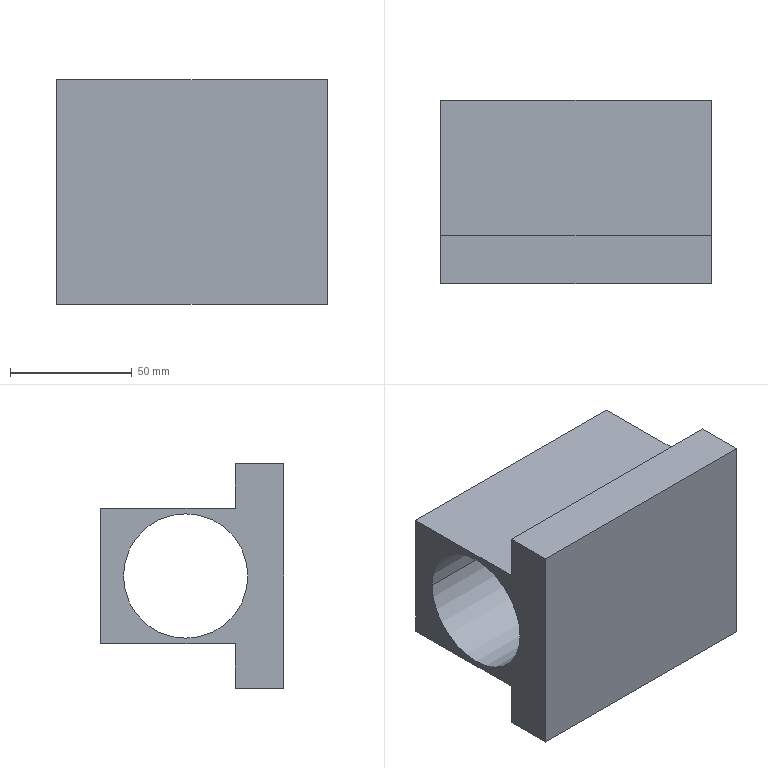Component | SolidWorks | ConnectingSeat-1 | 1 solid | 30 faces | box 111 x 75.24 x 92.14 mm | volume 314460 mm3 | plane 16 | cylinder 14 | commonest cylinder face diameters 8 x8 5.551 x4 51.14 x2
build123d program:
from build123d import *

# Parameters (mm, degrees)
BOSS_EXTRUDE1_DEPTH = 111
SKETCH4_R           = 18.564
CUT_EXTRUDE1_DEPTH  = 111
SKETCH5_W           = 55.24
SKETCH5_H           = 35.775
CUT_EXTRUDE2_DEPTH  = 171
SKETCH6_R           = 25.57
CUT_EXTRUDE3_DEPTH  = 115
SKETCH7_R           = 25.57
BOSS_EXTRUDE2_DEPTH = 111
SKETCH9_R           = 4
CUT_EXTRUDE4_DEPTH  = 13.5
SKETCH10_R          = 2.776
CUT_EXTRUDE5_DEPTH  = 13.5


with BuildPart() as part:
    # Sketch3 → Boss-Extrude1 (new body)
    with BuildSketch(Plane.ZY.offset(277)):
        Polygon((-20, -46.072), (-20, 46.072), (-0.1784, 46.072), (-0.1784, 27.887), (55.24, 27.887), (55.24, -27.887), (-0.1784, -27.887), (-0.1784, -46.072), align=None)
    extrude(amount=-BOSS_EXTRUDE1_DEPTH)

    # Sketch4 → Cut-Extrude1 (cut)
    with BuildSketch(Plane.ZY.offset(277)):
        with Locations((20.219, 0)):
            Circle(SKETCH4_R)
    extrude(amount=-CUT_EXTRUDE1_DEPTH, mode=Mode.SUBTRACT)

    # Sketch5 → Cut-Extrude2 (cut)
    with BuildSketch(Plane(origin=(-166, 0, 0), x_dir=(0, 0, -1), z_dir=(1, 0, 0))):
        with Locations((-17.62, 0)):
            Rectangle(SKETCH5_W, SKETCH5_H)
    extrude(amount=-CUT_EXTRUDE2_DEPTH, mode=Mode.SUBTRACT)

    # Sketch6 → Cut-Extrude3 (cut)
    with BuildSketch(Plane(origin=(-166, 0, 0), x_dir=(0, 0, -1), z_dir=(1, 0, 0))):
        with Locations((-20.219, 0)):
            Circle(SKETCH6_R)
    extrude(amount=-CUT_EXTRUDE3_DEPTH, mode=Mode.SUBTRACT)

    # Sketch7 → Boss-Extrude2 (add)
    with BuildSketch(Plane(origin=(-166, 0, 0), x_dir=(0, 0, -1), z_dir=(1, 0, 0))):
        Polygon((-55.24, 27.887), (-55.24, -27.887), (0.1784, -27.887), (0.1784, -46.072), (20, -46.072), (20, 46.072), (0.1784, 46.072), (0.1784, 27.887), align=None)
        with Locations((-20.219, 0)):
            Circle(SKETCH7_R, mode=Mode.SUBTRACT)
    extrude(amount=-BOSS_EXTRUDE2_DEPTH)

    # Sketch9 → Cut-Extrude4 (cut)
    with BuildSketch(Plane.XY.offset(-0.1784)):
        with Locations((-256.037, 36.566)):
            Circle(SKETCH9_R)
        with Locations((-186.382, 36.566)):
            Circle(SKETCH9_R)
        with Locations(Location((-186.382, -36.566, 0), (0, 0, 180))):
            Circle(SKETCH9_R)
        with Locations(Location((-256.037, -36.566, 0), (0, 0, 180))):
            Circle(SKETCH9_R)
    extrude(amount=-CUT_EXTRUDE4_DEPTH, mode=Mode.SUBTRACT)

    # Sketch10 → Cut-Extrude5 (cut)
    with BuildSketch(Plane.XY.offset(-0.1784)):
        with Locations((-221.326, 36.732)):
            Circle(SKETCH10_R)
        with Locations(Location((-221.326, -36.732, 0), (0, 0, 180))):
            Circle(SKETCH10_R)
    extrude(amount=-CUT_EXTRUDE5_DEPTH, mode=Mode.SUBTRACT)


solid = part.part

# Placed as in the assembly
solid = solid.moved(Location((0, 40, 0), (-90, 0, 0)))
STEP:
#1=CARTESIAN_POINT('',(-8.823,1.036,1.446));
#2=VERTEX_POINT('',#1);
#3=CARTESIAN_POINT('',(-8.604,1.036,1.446));
#4=VERTEX_POINT('',#3);
#5=CARTESIAN_POINT('',(-8.714,1.036,1.446));
#6=DIRECTION('',(0.,1.,0.));
#7=DIRECTION('',(-1.,0.,0.));
#8=AXIS2_PLACEMENT_3D('',#5,#6,#7);
#9=CIRCLE('',#8,0.1093);
#10=EDGE_CURVE('',#2,#4,#9,.T.);
#11=ORIENTED_EDGE('',*,*,#10,.F.);
#12=CARTESIAN_POINT('',(-8.823,1.568,1.446));
#13=VERTEX_POINT('',#12);
#14=CARTESIAN_POINT('',(-8.823,1.036,1.446));
#15=DIRECTION('',(0.,1.,0.));
#16=VECTOR('',#15,39.37);
#17=LINE('',#14,#16);
#18=EDGE_CURVE('',#2,#13,#17,.T.);
#19=ORIENTED_EDGE('',*,*,#18,.T.);
#20=CARTESIAN_POINT('',(-8.604,1.568,1.446));
#21=VERTEX_POINT('',#20);
#22=CARTESIAN_POINT('',(-8.714,1.568,1.446));
#23=DIRECTION('',(0.,1.,0.));
#24=DIRECTION('',(-1.,0.,0.));
#25=AXIS2_PLACEMENT_3D('',#22,#23,#24);
#26=CIRCLE('',#25,0.1093);
#27=EDGE_CURVE('',#13,#21,#26,.T.);
#28=ORIENTED_EDGE('',*,*,#27,.T.);
#29=CARTESIAN_POINT('',(-8.604,1.036,1.446));
#30=DIRECTION('',(0.,1.,0.));
#31=VECTOR('',#30,39.37);
#32=LINE('',#29,#31);
#33=EDGE_CURVE('',#4,#21,#32,.T.);
#34=ORIENTED_EDGE('',*,*,#33,.F.);
#35=EDGE_LOOP('',(#11,#19,#28,#34));
#36=FACE_OUTER_BOUND('',#35,.T.);
#37=CARTESIAN_POINT('',(-8.714,1.036,1.446));
#38=DIRECTION('',(0.,1.,0.));
#39=DIRECTION('',(1.,0.,0.));
#40=AXIS2_PLACEMENT_3D('',#37,#38,#39);
#41=CYLINDRICAL_SURFACE('',#40,0.1093);
#42=ADVANCED_FACE('',(#36),#41,.F.);
#43=CARTESIAN_POINT('',(-8.823,1.036,-1.446));
#44=VERTEX_POINT('',#43);
#45=CARTESIAN_POINT('',(-8.604,1.036,-1.446));
#46=VERTEX_POINT('',#45);
#47=CARTESIAN_POINT('',(-8.714,1.036,-1.446));
#48=DIRECTION('',(0.,1.,0.));
#49=DIRECTION('',(1.,0.,0.));
#50=AXIS2_PLACEMENT_3D('',#47,#48,#49);
#51=CIRCLE('',#50,0.1093);
#52=EDGE_CURVE('',#44,#46,#51,.T.);
#53=ORIENTED_EDGE('',*,*,#52,.F.);
#54=CARTESIAN_POINT('',(-8.823,1.568,-1.446));
#55=VERTEX_POINT('',#54);
#56=CARTESIAN_POINT('',(-8.823,1.036,-1.446));
#57=DIRECTION('',(0.,1.,0.));
#58=VECTOR('',#57,39.37);
#59=LINE('',#56,#58);
#60=EDGE_CURVE('',#44,#55,#59,.T.);
#61=ORIENTED_EDGE('',*,*,#60,.T.);
#62=CARTESIAN_POINT('',(-8.604,1.568,-1.446));
#63=VERTEX_POINT('',#62);
#64=CARTESIAN_POINT('',(-8.714,1.568,-1.446));
#65=DIRECTION('',(0.,1.,0.));
#66=DIRECTION('',(1.,0.,0.));
#67=AXIS2_PLACEMENT_3D('',#64,#65,#66);
#68=CIRCLE('',#67,0.1093);
#69=EDGE_CURVE('',#55,#63,#68,.T.);
#70=ORIENTED_EDGE('',*,*,#69,.T.);
#71=CARTESIAN_POINT('',(-8.604,1.036,-1.446));
#72=DIRECTION('',(0.,1.,0.));
#73=VECTOR('',#72,39.37);
#74=LINE('',#71,#73);
#75=EDGE_CURVE('',#46,#63,#74,.T.);
#76=ORIENTED_EDGE('',*,*,#75,.F.);
#77=EDGE_LOOP('',(#53,#61,#70,#76));
#78=FACE_OUTER_BOUND('',#77,.T.);
#79=CARTESIAN_POINT('',(-8.714,1.036,-1.446));
#80=DIRECTION('',(0.,1.,0.));
#81=DIRECTION('',(1.,0.,0.));
#82=AXIS2_PLACEMENT_3D('',#79,#80,#81);
#83=CYLINDRICAL_SURFACE('',#82,0.1093);
#84=ADVANCED_FACE('',(#78),#83,.F.);
#85=CARTESIAN_POINT('',(-10.238,1.036,1.44));
#86=VERTEX_POINT('',#85);
#87=CARTESIAN_POINT('',(-9.923,1.036,1.44));
#88=VERTEX_POINT('',#87);
#89=CARTESIAN_POINT('',(-10.08,1.036,1.44));
#90=DIRECTION('',(0.,1.,0.));
#91=DIRECTION('',(-1.,0.,0.));
#92=AXIS2_PLACEMENT_3D('',#89,#90,#91);
#93=CIRCLE('',#92,0.1575);
#94=EDGE_CURVE('',#86,#88,#93,.T.);
#95=ORIENTED_EDGE('',*,*,#94,.F.);
#96=CARTESIAN_POINT('',(-10.238,1.568,1.44));
#97=VERTEX_POINT('',#96);
#98=CARTESIAN_POINT('',(-10.238,1.036,1.44));
#99=DIRECTION('',(0.,1.,0.));
#100=VECTOR('',#99,39.37);
#101=LINE('',#98,#100);
#102=EDGE_CURVE('',#86,#97,#101,.T.);
#103=ORIENTED_EDGE('',*,*,#102,.T.);
#104=CARTESIAN_POINT('',(-9.923,1.568,1.44));
#105=VERTEX_POINT('',#104);
#106=CARTESIAN_POINT('',(-10.08,1.568,1.44));
#107=DIRECTION('',(0.,1.,0.));
#108=DIRECTION('',(-1.,0.,0.));
#109=AXIS2_PLACEMENT_3D('',#106,#107,#108);
#110=CIRCLE('',#109,0.1575);
#111=EDGE_CURVE('',#97,#105,#110,.T.);
#112=ORIENTED_EDGE('',*,*,#111,.T.);
#113=CARTESIAN_POINT('',(-9.923,1.036,1.44));
#114=DIRECTION('',(0.,1.,0.));
#115=VECTOR('',#114,39.37);
#116=LINE('',#113,#115);
#117=EDGE_CURVE('',#88,#105,#116,.T.);
#118=ORIENTED_EDGE('',*,*,#117,.F.);
#119=EDGE_LOOP('',(#95,#103,#112,#118));
#120=FACE_OUTER_BOUND('',#119,.T.);
#121=CARTESIAN_POINT('',(-10.08,1.036,1.44));
#122=DIRECTION('',(0.,1.,0.));
#123=DIRECTION('',(1.,0.,0.));
#124=AXIS2_PLACEMENT_3D('',#121,#122,#123);
#125=CYLINDRICAL_SURFACE('',#124,0.1575);
#126=ADVANCED_FACE('',(#120),#125,.F.);
#127=CARTESIAN_POINT('',(-7.495,1.036,1.44));
#128=VERTEX_POINT('',#127);
#129=CARTESIAN_POINT('',(-7.18,1.036,1.44));
#130=VERTEX_POINT('',#129);
#131=CARTESIAN_POINT('',(-7.338,1.036,1.44));
#132=DIRECTION('',(0.,1.,0.));
#133=DIRECTION('',(-1.,0.,0.));
#134=AXIS2_PLACEMENT_3D('',#131,#132,#133);
#135=CIRCLE('',#134,0.1575);
#136=EDGE_CURVE('',#128,#130,#135,.T.);
#137=ORIENTED_EDGE('',*,*,#136,.F.);
#138=CARTESIAN_POINT('',(-7.495,1.568,1.44));
#139=VERTEX_POINT('',#138);
#140=CARTESIAN_POINT('',(-7.495,1.036,1.44));
#141=DIRECTION('',(0.,1.,0.));
#142=VECTOR('',#141,39.37);
#143=LINE('',#140,#142);
#144=EDGE_CURVE('',#128,#139,#143,.T.);
#145=ORIENTED_EDGE('',*,*,#144,.T.);
#146=CARTESIAN_POINT('',(-7.18,1.568,1.44));
#147=VERTEX_POINT('',#146);
#148=CARTESIAN_POINT('',(-7.338,1.568,1.44));
#149=DIRECTION('',(0.,1.,0.));
#150=DIRECTION('',(-1.,0.,0.));
#151=AXIS2_PLACEMENT_3D('',#148,#149,#150);
#152=CIRCLE('',#151,0.1575);
#153=EDGE_CURVE('',#139,#147,#152,.T.);
#154=ORIENTED_EDGE('',*,*,#153,.T.);
#155=CARTESIAN_POINT('',(-7.18,1.036,1.44));
#156=DIRECTION('',(0.,1.,0.));
#157=VECTOR('',#156,39.37);
#158=LINE('',#155,#157);
#159=EDGE_CURVE('',#130,#147,#158,.T.);
#160=ORIENTED_EDGE('',*,*,#159,.F.);
#161=EDGE_LOOP('',(#137,#145,#154,#160));
#162=FACE_OUTER_BOUND('',#161,.T.);
#163=CARTESIAN_POINT('',(-7.338,1.036,1.44));
#164=DIRECTION('',(0.,1.,0.));
#165=DIRECTION('',(1.,0.,0.));
#166=AXIS2_PLACEMENT_3D('',#163,#164,#165);
#167=CYLINDRICAL_SURFACE('',#166,0.1575);
#168=ADVANCED_FACE('',(#162),#167,.F.);
#169=CARTESIAN_POINT('',(-7.495,1.036,-1.44));
#170=VERTEX_POINT('',#169);
#171=CARTESIAN_POINT('',(-7.18,1.036,-1.44));
#172=VERTEX_POINT('',#171);
#173=CARTESIAN_POINT('',(-7.338,1.036,-1.44));
#174=DIRECTION('',(0.,1.,0.));
#175=DIRECTION('',(1.,0.,0.));
#176=AXIS2_PLACEMENT_3D('',#173,#174,#175);
#177=CIRCLE('',#176,0.1575);
#178=EDGE_CURVE('',#170,#172,#177,.T.);
#179=ORIENTED_EDGE('',*,*,#178,.F.);
#180=CARTESIAN_POINT('',(-7.495,1.568,-1.44));
#181=VERTEX_POINT('',#180);
#182=CARTESIAN_POINT('',(-7.495,1.036,-1.44));
#183=DIRECTION('',(0.,1.,0.));
#184=VECTOR('',#183,39.37);
#185=LINE('',#182,#184);
#186=EDGE_CURVE('',#170,#181,#185,.T.);
#187=ORIENTED_EDGE('',*,*,#186,.T.);
#188=CARTESIAN_POINT('',(-7.18,1.568,-1.44));
#189=VERTEX_POINT('',#188);
#190=CARTESIAN_POINT('',(-7.338,1.568,-1.44));
#191=DIRECTION('',(0.,1.,0.));
#192=DIRECTION('',(1.,0.,0.));
#193=AXIS2_PLACEMENT_3D('',#190,#191,#192);
#194=CIRCLE('',#193,0.1575);
#195=EDGE_CURVE('',#181,#189,#194,.T.);
#196=ORIENTED_EDGE('',*,*,#195,.T.);
#197=CARTESIAN_POINT('',(-7.18,1.036,-1.44));
#198=DIRECTION('',(0.,1.,0.));
#199=VECTOR('',#198,39.37);
#200=LINE('',#197,#199);
#201=EDGE_CURVE('',#172,#189,#200,.T.);
#202=ORIENTED_EDGE('',*,*,#201,.F.);
#203=EDGE_LOOP('',(#179,#187,#196,#202));
#204=FACE_OUTER_BOUND('',#203,.T.);
#205=CARTESIAN_POINT('',(-7.338,1.036,-1.44));
#206=DIRECTION('',(0.,1.,0.));
#207=DIRECTION('',(1.,0.,0.));
#208=AXIS2_PLACEMENT_3D('',#205,#206,#207);
#209=CYLINDRICAL_SURFACE('',#208,0.1575);
#210=ADVANCED_FACE('',(#204),#209,.F.);
#211=CARTESIAN_POINT('',(-10.238,1.036,-1.44));
#212=VERTEX_POINT('',#211);
#213=CARTESIAN_POINT('',(-9.923,1.036,-1.44));
#214=VERTEX_POINT('',#213);
#215=CARTESIAN_POINT('',(-10.08,1.036,-1.44));
#216=DIRECTION('',(0.,1.,0.));
#217=DIRECTION('',(1.,0.,0.));
#218=AXIS2_PLACEMENT_3D('',#215,#216,#217);
#219=CIRCLE('',#218,0.1575);
#220=EDGE_CURVE('',#212,#214,#219,.T.);
#221=ORIENTED_EDGE('',*,*,#220,.F.);
#222=CARTESIAN_POINT('',(-10.238,1.568,-1.44));
#223=VERTEX_POINT('',#222);
#224=CARTESIAN_POINT('',(-10.238,1.036,-1.44));
#225=DIRECTION('',(0.,1.,0.));
#226=VECTOR('',#225,39.37);
#227=LINE('',#224,#226);
#228=EDGE_CURVE('',#212,#223,#227,.T.);
#229=ORIENTED_EDGE('',*,*,#228,.T.);
#230=CARTESIAN_POINT('',(-9.923,1.568,-1.44));
#231=VERTEX_POINT('',#230);
#232=CARTESIAN_POINT('',(-10.08,1.568,-1.44));
#233=DIRECTION('',(0.,1.,0.));
#234=DIRECTION('',(1.,0.,0.));
#235=AXIS2_PLACEMENT_3D('',#232,#233,#234);
#236=CIRCLE('',#235,0.1575);
#237=EDGE_CURVE('',#223,#231,#236,.T.);
#238=ORIENTED_EDGE('',*,*,#237,.T.);
#239=CARTESIAN_POINT('',(-9.923,1.036,-1.44));
#240=DIRECTION('',(0.,1.,0.));
#241=VECTOR('',#240,39.37);
#242=LINE('',#239,#241);
#243=EDGE_CURVE('',#214,#231,#242,.T.);
#244=ORIENTED_EDGE('',*,*,#243,.F.);
#245=EDGE_LOOP('',(#221,#229,#238,#244));
#246=FACE_OUTER_BOUND('',#245,.T.);
#247=CARTESIAN_POINT('',(-10.08,1.036,-1.44));
#248=DIRECTION('',(0.,1.,0.));
#249=DIRECTION('',(1.,0.,0.));
#250=AXIS2_PLACEMENT_3D('',#247,#248,#249);
#251=CYLINDRICAL_SURFACE('',#250,0.1575);
#252=ADVANCED_FACE('',(#246),#251,.F.);
#253=CARTESIAN_POINT('',(-10.906,1.364,0.));
#254=VERTEX_POINT('',#253);
#255=CARTESIAN_POINT('',(-10.906,3.378,0.));
#256=VERTEX_POINT('',#255);
#257=CARTESIAN_POINT('',(-10.906,2.371,0.));
#258=DIRECTION('',(-1.,0.,0.));
#259=DIRECTION('',(0.,1.,0.));
#260=AXIS2_PLACEMENT_3D('',#257,#258,#259);
#261=CIRCLE('',#260,1.007);
#262=EDGE_CURVE('',#254,#256,#261,.T.);
#263=ORIENTED_EDGE('',*,*,#262,.T.);
#264=CARTESIAN_POINT('',(-6.535,3.378,0.));
#265=VERTEX_POINT('',#264);
#266=CARTESIAN_POINT('',(-11.063,3.378,0.));
#267=DIRECTION('',(1.,0.,0.));
#268=VECTOR('',#267,39.37);
#269=LINE('',#266,#268);
#270=EDGE_CURVE('',#256,#265,#269,.T.);
#271=ORIENTED_EDGE('',*,*,#270,.T.);
#272=CARTESIAN_POINT('',(-6.535,1.364,0.));
#273=VERTEX_POINT('',#272);
#274=CARTESIAN_POINT('',(-6.535,2.371,0.));
#275=DIRECTION('',(1.,0.,0.));
#276=DIRECTION('',(0.,-1.,0.));
#277=AXIS2_PLACEMENT_3D('',#274,#275,#276);
#278=CIRCLE('',#277,1.007);
#279=EDGE_CURVE('',#265,#273,#278,.T.);
#280=ORIENTED_EDGE('',*,*,#279,.T.);
#281=CARTESIAN_POINT('',(-11.063,1.364,0.));
#282=DIRECTION('',(1.,0.,0.));
#283=VECTOR('',#282,39.37);
#284=LINE('',#281,#283);
#285=EDGE_CURVE('',#254,#273,#284,.T.);
#286=ORIENTED_EDGE('',*,*,#285,.F.);
#287=EDGE_LOOP('',(#263,#271,#280,#286));
#288=FACE_OUTER_BOUND('',#287,.T.);
#289=CARTESIAN_POINT('',(-11.063,2.371,0.));
#290=DIRECTION('',(1.,0.,0.));
#291=DIRECTION('',(0.,-1.,0.));
#292=AXIS2_PLACEMENT_3D('',#289,#290,#291);
#293=CYLINDRICAL_SURFACE('',#292,1.007);
#294=ADVANCED_FACE('',(#288),#293,.F.);
#295=CARTESIAN_POINT('',(-10.906,3.75,1.098));
#296=VERTEX_POINT('',#295);
#297=CARTESIAN_POINT('',(-10.906,3.75,-1.098));
#298=VERTEX_POINT('',#297);
#299=CARTESIAN_POINT('',(-10.906,3.75,-1.098));
#300=DIRECTION('',(0.,0.,-1.));
#301=VECTOR('',#300,39.37);
#302=LINE('',#299,#301);
#303=EDGE_CURVE('',#296,#298,#302,.T.);
#304=ORIENTED_EDGE('',*,*,#303,.F.);
#305=CARTESIAN_POINT('',(-6.535,3.75,1.098));
#306=VERTEX_POINT('',#305);
#307=CARTESIAN_POINT('',(-6.535,3.75,1.098));
#308=DIRECTION('',(-1.,0.,0.));
#309=VECTOR('',#308,39.37);
#310=LINE('',#307,#309);
#311=EDGE_CURVE('',#306,#296,#310,.T.);
#312=ORIENTED_EDGE('',*,*,#311,.F.);
#313=CARTESIAN_POINT('',(-6.535,3.75,-1.098));
#314=VERTEX_POINT('',#313);
#315=CARTESIAN_POINT('',(-6.535,3.75,-1.098));
#316=DIRECTION('',(0.,0.,-1.));
#317=VECTOR('',#316,39.37);
#318=LINE('',#315,#317);
#319=EDGE_CURVE('',#306,#314,#318,.T.);
#320=ORIENTED_EDGE('',*,*,#319,.T.);
#321=CARTESIAN_POINT('',(-6.535,3.75,-1.098));
#322=DIRECTION('',(-1.,0.,0.));
#323=VECTOR('',#322,39.37);
#324=LINE('',#321,#323);
#325=EDGE_CURVE('',#314,#298,#324,.T.);
#326=ORIENTED_EDGE('',*,*,#325,.T.);
#327=EDGE_LOOP('',(#304,#312,#320,#326));
#328=FACE_OUTER_BOUND('',#327,.T.);
#329=CARTESIAN_POINT('',(-6.535,3.75,-1.098));
#330=DIRECTION('',(0.,1.,0.));
#331=DIRECTION('',(1.,0.,0.));
#332=AXIS2_PLACEMENT_3D('',#329,#330,#331);
#333=PLANE('',#332);
#334=ADVANCED_FACE('',(#328),#333,.T.);
#335=CARTESIAN_POINT('',(-10.906,1.568,1.098));
#336=VERTEX_POINT('',#335);
#337=CARTESIAN_POINT('',(-10.906,1.568,1.098));
#338=DIRECTION('',(0.,1.,0.));
#339=VECTOR('',#338,39.37);
#340=LINE('',#337,#339);
#341=EDGE_CURVE('',#336,#296,#340,.T.);
#342=ORIENTED_EDGE('',*,*,#341,.F.);
#343=CARTESIAN_POINT('',(-6.535,1.568,1.098));
#344=VERTEX_POINT('',#343);
#345=CARTESIAN_POINT('',(-6.535,1.568,1.098));
#346=DIRECTION('',(-1.,0.,0.));
#347=VECTOR('',#346,39.37);
#348=LINE('',#345,#347);
#349=EDGE_CURVE('',#344,#336,#348,.T.);
#350=ORIENTED_EDGE('',*,*,#349,.F.);
#351=CARTESIAN_POINT('',(-6.535,1.568,1.098));
#352=DIRECTION('',(0.,1.,0.));
#353=VECTOR('',#352,39.37);
#354=LINE('',#351,#353);
#355=EDGE_CURVE('',#344,#306,#354,.T.);
#356=ORIENTED_EDGE('',*,*,#355,.T.);
#357=ORIENTED_EDGE('',*,*,#311,.T.);
#358=EDGE_LOOP('',(#342,#350,#356,#357));
#359=FACE_OUTER_BOUND('',#358,.T.);
#360=CARTESIAN_POINT('',(-6.535,1.568,1.098));
#361=DIRECTION('',(0.,0.,1.));
#362=DIRECTION('',(0.,-1.,0.));
#363=AXIS2_PLACEMENT_3D('',#360,#361,#362);
#364=PLANE('',#363);
#365=ADVANCED_FACE('',(#359),#364,.T.);
#366=CARTESIAN_POINT('',(-8.714,1.568,1.446));
#367=DIRECTION('',(0.,1.,0.));
#368=DIRECTION('',(-1.,0.,0.));
#369=AXIS2_PLACEMENT_3D('',#366,#367,#368);
#370=CIRCLE('',#369,0.1093);
#371=EDGE_CURVE('',#21,#13,#370,.T.);
#372=ORIENTED_EDGE('',*,*,#371,.F.);
#373=ORIENTED_EDGE('',*,*,#27,.F.);
#374=EDGE_LOOP('',(#372,#373));
#375=FACE_BOUND('',#374,.T.);
#376=CARTESIAN_POINT('',(-10.08,1.568,1.44));
#377=DIRECTION('',(0.,1.,0.));
#378=DIRECTION('',(-1.,0.,0.));
#379=AXIS2_PLACEMENT_3D('',#376,#377,#378);
#380=CIRCLE('',#379,0.1575);
#381=EDGE_CURVE('',#105,#97,#380,.T.);
#382=ORIENTED_EDGE('',*,*,#381,.F.);
#383=ORIENTED_EDGE('',*,*,#111,.F.);
#384=EDGE_LOOP('',(#382,#383));
#385=FACE_BOUND('',#384,.T.);
#386=CARTESIAN_POINT('',(-7.338,1.568,1.44));
#387=DIRECTION('',(0.,1.,0.));
#388=DIRECTION('',(-1.,0.,0.));
#389=AXIS2_PLACEMENT_3D('',#386,#387,#388);
#390=CIRCLE('',#389,0.1575);
#391=EDGE_CURVE('',#147,#139,#390,.T.);
#392=ORIENTED_EDGE('',*,*,#391,.F.);
#393=ORIENTED_EDGE('',*,*,#153,.F.);
#394=EDGE_LOOP('',(#392,#393));
#395=FACE_BOUND('',#394,.T.);
#396=CARTESIAN_POINT('',(-10.906,1.568,1.814));
#397=VERTEX_POINT('',#396);
#398=CARTESIAN_POINT('',(-10.906,1.568,1.814));
#399=DIRECTION('',(0.,0.,-1.));
#400=VECTOR('',#399,39.37);
#401=LINE('',#398,#400);
#402=EDGE_CURVE('',#397,#336,#401,.T.);
#403=ORIENTED_EDGE('',*,*,#402,.F.);
#404=CARTESIAN_POINT('',(-6.535,1.568,1.814));
#405=VERTEX_POINT('',#404);
#406=CARTESIAN_POINT('',(-6.535,1.568,1.814));
#407=DIRECTION('',(-1.,0.,0.));
#408=VECTOR('',#407,39.37);
#409=LINE('',#406,#408);
#410=EDGE_CURVE('',#405,#397,#409,.T.);
#411=ORIENTED_EDGE('',*,*,#410,.F.);
#412=CARTESIAN_POINT('',(-6.535,1.568,1.814));
#413=DIRECTION('',(0.,0.,-1.));
#414=VECTOR('',#413,39.37);
#415=LINE('',#412,#414);
#416=EDGE_CURVE('',#405,#344,#415,.T.);
#417=ORIENTED_EDGE('',*,*,#416,.T.);
#418=ORIENTED_EDGE('',*,*,#349,.T.);
#419=EDGE_LOOP('',(#403,#411,#417,#418));
#420=FACE_OUTER_BOUND('',#419,.T.);
#421=CARTESIAN_POINT('',(-6.535,1.568,1.814));
#422=DIRECTION('',(0.,1.,0.));
#423=DIRECTION('',(0.,-0.,1.));
#424=AXIS2_PLACEMENT_3D('',#421,#422,#423);
#425=PLANE('',#424);
#426=ADVANCED_FACE('',(#375,#385,#395,#420),#425,.T.);
#427=CARTESIAN_POINT('',(-10.906,0.7874,1.814));
#428=VERTEX_POINT('',#427);
#429=CARTESIAN_POINT('',(-10.906,0.7874,1.814));
#430=DIRECTION('',(0.,1.,0.));
#431=VECTOR('',#430,39.37);
#432=LINE('',#429,#431);
#433=EDGE_CURVE('',#428,#397,#432,.T.);
#434=ORIENTED_EDGE('',*,*,#433,.F.);
#435=CARTESIAN_POINT('',(-6.535,0.7874,1.814));
#436=VERTEX_POINT('',#435);
#437=CARTESIAN_POINT('',(-6.535,0.7874,1.814));
#438=DIRECTION('',(-1.,0.,0.));
#439=VECTOR('',#438,39.37);
#440=LINE('',#437,#439);
#441=EDGE_CURVE('',#436,#428,#440,.T.);
#442=ORIENTED_EDGE('',*,*,#441,.F.);
#443=CARTESIAN_POINT('',(-6.535,0.7874,1.814));
#444=DIRECTION('',(0.,1.,0.));
#445=VECTOR('',#444,39.37);
#446=LINE('',#443,#445);
#447=EDGE_CURVE('',#436,#405,#446,.T.);
#448=ORIENTED_EDGE('',*,*,#447,.T.);
#449=ORIENTED_EDGE('',*,*,#410,.T.);
#450=EDGE_LOOP('',(#434,#442,#448,#449));
#451=FACE_OUTER_BOUND('',#450,.T.);
#452=CARTESIAN_POINT('',(-6.535,0.7874,1.814));
#453=DIRECTION('',(0.,-0.,1.));
#454=DIRECTION('',(0.,-1.,-0.));
#455=AXIS2_PLACEMENT_3D('',#452,#453,#454);
#456=PLANE('',#455);
#457=ADVANCED_FACE('',(#451),#456,.T.);
#458=CARTESIAN_POINT('',(-10.906,0.7874,-1.814));
#459=VERTEX_POINT('',#458);
#460=CARTESIAN_POINT('',(-10.906,0.7874,1.814));
#461=DIRECTION('',(0.,-0.,1.));
#462=VECTOR('',#461,39.37);
#463=LINE('',#460,#462);
#464=EDGE_CURVE('',#459,#428,#463,.T.);
#465=ORIENTED_EDGE('',*,*,#464,.F.);
#466=CARTESIAN_POINT('',(-6.535,0.7874,-1.814));
#467=VERTEX_POINT('',#466);
#468=CARTESIAN_POINT('',(-6.535,0.7874,-1.814));
#469=DIRECTION('',(-1.,0.,0.));
#470=VECTOR('',#469,39.37);
#471=LINE('',#468,#470);
#472=EDGE_CURVE('',#467,#459,#471,.T.);
#473=ORIENTED_EDGE('',*,*,#472,.F.);
#474=CARTESIAN_POINT('',(-6.535,0.7874,1.814));
#475=DIRECTION('',(0.,-0.,1.));
#476=VECTOR('',#475,39.37);
#477=LINE('',#474,#476);
#478=EDGE_CURVE('',#467,#436,#477,.T.);
#479=ORIENTED_EDGE('',*,*,#478,.T.);
#480=ORIENTED_EDGE('',*,*,#441,.T.);
#481=EDGE_LOOP('',(#465,#473,#479,#480));
#482=FACE_OUTER_BOUND('',#481,.T.);
#483=CARTESIAN_POINT('',(-6.535,0.7874,1.814));
#484=DIRECTION('',(0.,-1.,-0.));
#485=DIRECTION('',(0.,0.,-1.));
#486=AXIS2_PLACEMENT_3D('',#483,#484,#485);
#487=PLANE('',#486);
#488=ADVANCED_FACE('',(#482),#487,.T.);
#489=CARTESIAN_POINT('',(-10.906,1.568,-1.814));
#490=VERTEX_POINT('',#489);
#491=CARTESIAN_POINT('',(-10.906,0.7874,-1.814));
#492=DIRECTION('',(0.,-1.,0.));
#493=VECTOR('',#492,39.37);
#494=LINE('',#491,#493);
#495=EDGE_CURVE('',#490,#459,#494,.T.);
#496=ORIENTED_EDGE('',*,*,#495,.F.);
#497=CARTESIAN_POINT('',(-6.535,1.568,-1.814));
#498=VERTEX_POINT('',#497);
#499=CARTESIAN_POINT('',(-6.535,1.568,-1.814));
#500=DIRECTION('',(-1.,0.,0.));
#501=VECTOR('',#500,39.37);
#502=LINE('',#499,#501);
#503=EDGE_CURVE('',#498,#490,#502,.T.);
#504=ORIENTED_EDGE('',*,*,#503,.F.);
#505=CARTESIAN_POINT('',(-6.535,0.7874,-1.814));
#506=DIRECTION('',(0.,-1.,0.));
#507=VECTOR('',#506,39.37);
#508=LINE('',#505,#507);
#509=EDGE_CURVE('',#498,#467,#508,.T.);
#510=ORIENTED_EDGE('',*,*,#509,.T.);
#511=ORIENTED_EDGE('',*,*,#472,.T.);
#512=EDGE_LOOP('',(#496,#504,#510,#511));
#513=FACE_OUTER_BOUND('',#512,.T.);
#514=CARTESIAN_POINT('',(-6.535,0.7874,-1.814));
#515=DIRECTION('',(0.,0.,-1.));
#516=DIRECTION('',(0.,1.,0.));
#517=AXIS2_PLACEMENT_3D('',#514,#515,#516);
#518=PLANE('',#517);
#519=ADVANCED_FACE('',(#513),#518,.T.);
#520=CARTESIAN_POINT('',(-8.714,1.568,-1.446));
#521=DIRECTION('',(0.,1.,0.));
#522=DIRECTION('',(1.,0.,0.));
#523=AXIS2_PLACEMENT_3D('',#520,#521,#522);
#524=CIRCLE('',#523,0.1093);
#525=EDGE_CURVE('',#63,#55,#524,.T.);
#526=ORIENTED_EDGE('',*,*,#525,.F.);
#527=ORIENTED_EDGE('',*,*,#69,.F.);
#528=EDGE_LOOP('',(#526,#527));
#529=FACE_BOUND('',#528,.T.);
#530=CARTESIAN_POINT('',(-7.338,1.568,-1.44));
#531=DIRECTION('',(0.,1.,0.));
#532=DIRECTION('',(1.,0.,0.));
#533=AXIS2_PLACEMENT_3D('',#530,#531,#532);
#534=CIRCLE('',#533,0.1575);
#535=EDGE_CURVE('',#189,#181,#534,.T.);
#536=ORIENTED_EDGE('',*,*,#535,.F.);
#537=ORIENTED_EDGE('',*,*,#195,.F.);
#538=EDGE_LOOP('',(#536,#537));
#539=FACE_BOUND('',#538,.T.);
#540=CARTESIAN_POINT('',(-10.08,1.568,-1.44));
#541=DIRECTION('',(0.,1.,0.));
#542=DIRECTION('',(1.,0.,0.));
#543=AXIS2_PLACEMENT_3D('',#540,#541,#542);
#544=CIRCLE('',#543,0.1575);
#545=EDGE_CURVE('',#231,#223,#544,.T.);
#546=ORIENTED_EDGE('',*,*,#545,.F.);
#547=ORIENTED_EDGE('',*,*,#237,.F.);
#548=EDGE_LOOP('',(#546,#547));
#549=FACE_BOUND('',#548,.T.);
#550=CARTESIAN_POINT('',(-10.906,1.568,-1.098));
#551=VERTEX_POINT('',#550);
#552=CARTESIAN_POINT('',(-10.906,1.568,-1.814));
#553=DIRECTION('',(0.,0.,-1.));
#554=VECTOR('',#553,39.37);
#555=LINE('',#552,#554);
#556=EDGE_CURVE('',#551,#490,#555,.T.);
#557=ORIENTED_EDGE('',*,*,#556,.F.);
#558=CARTESIAN_POINT('',(-6.535,1.568,-1.098));
#559=VERTEX_POINT('',#558);
#560=CARTESIAN_POINT('',(-6.535,1.568,-1.098));
#561=DIRECTION('',(-1.,0.,0.));
#562=VECTOR('',#561,39.37);
#563=LINE('',#560,#562);
#564=EDGE_CURVE('',#559,#551,#563,.T.);
#565=ORIENTED_EDGE('',*,*,#564,.F.);
#566=CARTESIAN_POINT('',(-6.535,1.568,-1.814));
#567=DIRECTION('',(0.,0.,-1.));
#568=VECTOR('',#567,39.37);
#569=LINE('',#566,#568);
#570=EDGE_CURVE('',#559,#498,#569,.T.);
#571=ORIENTED_EDGE('',*,*,#570,.T.);
#572=ORIENTED_EDGE('',*,*,#503,.T.);
#573=EDGE_LOOP('',(#557,#565,#571,#572));
#574=FACE_OUTER_BOUND('',#573,.T.);
#575=CARTESIAN_POINT('',(-6.535,1.568,-1.814));
#576=DIRECTION('',(0.,1.,0.));
#577=DIRECTION('',(1.,0.,0.));
#578=AXIS2_PLACEMENT_3D('',#575,#576,#577);
#579=PLANE('',#578);
#580=ADVANCED_FACE('',(#529,#539,#549,#574),#579,.T.);
#581=CARTESIAN_POINT('',(-10.906,1.568,-1.098));
#582=DIRECTION('',(0.,-1.,0.));
#583=VECTOR('',#582,39.37);
#584=LINE('',#581,#583);
#585=EDGE_CURVE('',#298,#551,#584,.T.);
#586=ORIENTED_EDGE('',*,*,#585,.F.);
#587=ORIENTED_EDGE('',*,*,#325,.F.);
#588=CARTESIAN_POINT('',(-6.535,1.568,-1.098));
#589=DIRECTION('',(0.,-1.,0.));
#590=VECTOR('',#589,39.37);
#591=LINE('',#588,#590);
#592=EDGE_CURVE('',#314,#559,#591,.T.);
#593=ORIENTED_EDGE('',*,*,#592,.T.);
#594=ORIENTED_EDGE('',*,*,#564,.T.);
#595=EDGE_LOOP('',(#586,#587,#593,#594));
#596=FACE_OUTER_BOUND('',#595,.T.);
#597=CARTESIAN_POINT('',(-6.535,1.568,-1.098));
#598=DIRECTION('',(0.,0.,-1.));
#599=DIRECTION('',(0.,1.,0.));
#600=AXIS2_PLACEMENT_3D('',#597,#598,#599);
#601=PLANE('',#600);
#602=ADVANCED_FACE('',(#596),#601,.T.);
#603=CARTESIAN_POINT('',(-6.535,2.371,0.));
#604=DIRECTION('',(1.,0.,0.));
#605=DIRECTION('',(0.,-1.,0.));
#606=AXIS2_PLACEMENT_3D('',#603,#604,#605);
#607=CIRCLE('',#606,1.007);
#608=EDGE_CURVE('',#273,#265,#607,.T.);
#609=ORIENTED_EDGE('',*,*,#608,.F.);
#610=ORIENTED_EDGE('',*,*,#279,.F.);
#611=EDGE_LOOP('',(#609,#610));
#612=FACE_BOUND('',#611,.T.);
#613=ORIENTED_EDGE('',*,*,#319,.F.);
#614=ORIENTED_EDGE('',*,*,#355,.F.);
#615=ORIENTED_EDGE('',*,*,#416,.F.);
#616=ORIENTED_EDGE('',*,*,#447,.F.);
#617=ORIENTED_EDGE('',*,*,#478,.F.);
#618=ORIENTED_EDGE('',*,*,#509,.F.);
#619=ORIENTED_EDGE('',*,*,#570,.F.);
#620=ORIENTED_EDGE('',*,*,#592,.F.);
#621=EDGE_LOOP('',(#613,#614,#615,#616,#617,#618,#619,#620));
#622=FACE_OUTER_BOUND('',#621,.T.);
#623=CARTESIAN_POINT('',(-6.535,1.575,0.));
#624=DIRECTION('',(-1.,0.,0.));
#625=DIRECTION('',(0.,1.,0.));
#626=AXIS2_PLACEMENT_3D('',#623,#624,#625);
#627=PLANE('',#626);
#628=ADVANCED_FACE('',(#612,#622),#627,.F.);
#629=ORIENTED_EDGE('',*,*,#262,.F.);
#630=CARTESIAN_POINT('',(-10.906,2.371,0.));
#631=DIRECTION('',(-1.,0.,0.));
#632=DIRECTION('',(0.,1.,0.));
#633=AXIS2_PLACEMENT_3D('',#630,#631,#632);
#634=CIRCLE('',#633,1.007);
#635=EDGE_CURVE('',#256,#254,#634,.T.);
#636=ORIENTED_EDGE('',*,*,#635,.F.);
#637=EDGE_LOOP('',(#629,#636));
#638=FACE_BOUND('',#637,.T.);
#639=ORIENTED_EDGE('',*,*,#303,.T.);
#640=ORIENTED_EDGE('',*,*,#585,.T.);
#641=ORIENTED_EDGE('',*,*,#556,.T.);
#642=ORIENTED_EDGE('',*,*,#495,.T.);
#643=ORIENTED_EDGE('',*,*,#464,.T.);
#644=ORIENTED_EDGE('',*,*,#433,.T.);
#645=ORIENTED_EDGE('',*,*,#402,.T.);
#646=ORIENTED_EDGE('',*,*,#341,.T.);
#647=EDGE_LOOP('',(#639,#640,#641,#642,#643,#644,#645,#646));
#648=FACE_OUTER_BOUND('',#647,.T.);
#649=CARTESIAN_POINT('',(-10.906,1.575,0.));
#650=DIRECTION('',(-1.,0.,0.));
#651=DIRECTION('',(0.,1.,0.));
#652=AXIS2_PLACEMENT_3D('',#649,#650,#651);
#653=PLANE('',#652);
#654=ADVANCED_FACE('',(#638,#648),#653,.T.);
#655=ORIENTED_EDGE('',*,*,#270,.F.);
#656=ORIENTED_EDGE('',*,*,#635,.T.);
#657=ORIENTED_EDGE('',*,*,#285,.T.);
#658=ORIENTED_EDGE('',*,*,#608,.T.);
#659=EDGE_LOOP('',(#655,#656,#657,#658));
#660=FACE_OUTER_BOUND('',#659,.T.);
#661=CARTESIAN_POINT('',(-11.063,2.371,0.));
#662=DIRECTION('',(1.,0.,0.));
#663=DIRECTION('',(0.,-1.,0.));
#664=AXIS2_PLACEMENT_3D('',#661,#662,#663);
#665=CYLINDRICAL_SURFACE('',#664,1.007);
#666=ADVANCED_FACE('',(#660),#665,.F.);
#667=ORIENTED_EDGE('',*,*,#228,.F.);
#668=CARTESIAN_POINT('',(-10.08,1.036,-1.44));
#669=DIRECTION('',(0.,1.,0.));
#670=DIRECTION('',(1.,0.,0.));
#671=AXIS2_PLACEMENT_3D('',#668,#669,#670);
#672=CIRCLE('',#671,0.1575);
#673=EDGE_CURVE('',#214,#212,#672,.T.);
#674=ORIENTED_EDGE('',*,*,#673,.F.);
#675=ORIENTED_EDGE('',*,*,#243,.T.);
#676=ORIENTED_EDGE('',*,*,#545,.T.);
#677=EDGE_LOOP('',(#667,#674,#675,#676));
#678=FACE_OUTER_BOUND('',#677,.T.);
#679=CARTESIAN_POINT('',(-10.08,1.036,-1.44));
#680=DIRECTION('',(0.,1.,0.));
#681=DIRECTION('',(1.,0.,0.));
#682=AXIS2_PLACEMENT_3D('',#679,#680,#681);
#683=CYLINDRICAL_SURFACE('',#682,0.1575);
#684=ADVANCED_FACE('',(#678),#683,.F.);
#685=ORIENTED_EDGE('',*,*,#673,.T.);
#686=ORIENTED_EDGE('',*,*,#220,.T.);
#687=EDGE_LOOP('',(#685,#686));
#688=FACE_OUTER_BOUND('',#687,.T.);
#689=CARTESIAN_POINT('',(-10.08,1.036,-1.44));
#690=DIRECTION('',(0.,1.,0.));
#691=DIRECTION('',(1.,0.,0.));
#692=AXIS2_PLACEMENT_3D('',#689,#690,#691);
#693=PLANE('',#692);
#694=ADVANCED_FACE('',(#688),#693,.T.);
#695=ORIENTED_EDGE('',*,*,#186,.F.);
#696=CARTESIAN_POINT('',(-7.338,1.036,-1.44));
#697=DIRECTION('',(0.,1.,0.));
#698=DIRECTION('',(1.,0.,0.));
#699=AXIS2_PLACEMENT_3D('',#696,#697,#698);
#700=CIRCLE('',#699,0.1575);
#701=EDGE_CURVE('',#172,#170,#700,.T.);
#702=ORIENTED_EDGE('',*,*,#701,.F.);
#703=ORIENTED_EDGE('',*,*,#201,.T.);
#704=ORIENTED_EDGE('',*,*,#535,.T.);
#705=EDGE_LOOP('',(#695,#702,#703,#704));
#706=FACE_OUTER_BOUND('',#705,.T.);
#707=CARTESIAN_POINT('',(-7.338,1.036,-1.44));
#708=DIRECTION('',(0.,1.,0.));
#709=DIRECTION('',(1.,0.,0.));
#710=AXIS2_PLACEMENT_3D('',#707,#708,#709);
#711=CYLINDRICAL_SURFACE('',#710,0.1575);
#712=ADVANCED_FACE('',(#706),#711,.F.);
#713=ORIENTED_EDGE('',*,*,#701,.T.);
#714=ORIENTED_EDGE('',*,*,#178,.T.);
#715=EDGE_LOOP('',(#713,#714));
#716=FACE_OUTER_BOUND('',#715,.T.);
#717=CARTESIAN_POINT('',(-7.338,1.036,-1.44));
#718=DIRECTION('',(0.,1.,0.));
#719=DIRECTION('',(1.,0.,0.));
#720=AXIS2_PLACEMENT_3D('',#717,#718,#719);
#721=PLANE('',#720);
#722=ADVANCED_FACE('',(#716),#721,.T.);
#723=ORIENTED_EDGE('',*,*,#144,.F.);
#724=CARTESIAN_POINT('',(-7.338,1.036,1.44));
#725=DIRECTION('',(0.,1.,0.));
#726=DIRECTION('',(-1.,0.,0.));
#727=AXIS2_PLACEMENT_3D('',#724,#725,#726);
#728=CIRCLE('',#727,0.1575);
#729=EDGE_CURVE('',#130,#128,#728,.T.);
#730=ORIENTED_EDGE('',*,*,#729,.F.);
#731=ORIENTED_EDGE('',*,*,#159,.T.);
#732=ORIENTED_EDGE('',*,*,#391,.T.);
#733=EDGE_LOOP('',(#723,#730,#731,#732));
#734=FACE_OUTER_BOUND('',#733,.T.);
#735=CARTESIAN_POINT('',(-7.338,1.036,1.44));
#736=DIRECTION('',(0.,1.,0.));
#737=DIRECTION('',(1.,0.,0.));
#738=AXIS2_PLACEMENT_3D('',#735,#736,#737);
#739=CYLINDRICAL_SURFACE('',#738,0.1575);
#740=ADVANCED_FACE('',(#734),#739,.F.);
#741=ORIENTED_EDGE('',*,*,#729,.T.);
#742=ORIENTED_EDGE('',*,*,#136,.T.);
#743=EDGE_LOOP('',(#741,#742));
#744=FACE_OUTER_BOUND('',#743,.T.);
#745=CARTESIAN_POINT('',(-7.338,1.036,1.44));
#746=DIRECTION('',(0.,-1.,0.));
#747=DIRECTION('',(-1.,0.,0.));
#748=AXIS2_PLACEMENT_3D('',#745,#746,#747);
#749=PLANE('',#748);
#750=ADVANCED_FACE('',(#744),#749,.F.);
#751=ORIENTED_EDGE('',*,*,#102,.F.);
#752=CARTESIAN_POINT('',(-10.08,1.036,1.44));
#753=DIRECTION('',(0.,1.,0.));
#754=DIRECTION('',(-1.,0.,0.));
#755=AXIS2_PLACEMENT_3D('',#752,#753,#754);
#756=CIRCLE('',#755,0.1575);
#757=EDGE_CURVE('',#88,#86,#756,.T.);
#758=ORIENTED_EDGE('',*,*,#757,.F.);
#759=ORIENTED_EDGE('',*,*,#117,.T.);
#760=ORIENTED_EDGE('',*,*,#381,.T.);
#761=EDGE_LOOP('',(#751,#758,#759,#760));
#762=FACE_OUTER_BOUND('',#761,.T.);
#763=CARTESIAN_POINT('',(-10.08,1.036,1.44));
#764=DIRECTION('',(0.,1.,0.));
#765=DIRECTION('',(1.,0.,0.));
#766=AXIS2_PLACEMENT_3D('',#763,#764,#765);
#767=CYLINDRICAL_SURFACE('',#766,0.1575);
#768=ADVANCED_FACE('',(#762),#767,.F.);
#769=ORIENTED_EDGE('',*,*,#757,.T.);
#770=ORIENTED_EDGE('',*,*,#94,.T.);
#771=EDGE_LOOP('',(#769,#770));
#772=FACE_OUTER_BOUND('',#771,.T.);
#773=CARTESIAN_POINT('',(-10.08,1.036,1.44));
#774=DIRECTION('',(0.,-1.,0.));
#775=DIRECTION('',(-1.,0.,0.));
#776=AXIS2_PLACEMENT_3D('',#773,#774,#775);
#777=PLANE('',#776);
#778=ADVANCED_FACE('',(#772),#777,.F.);
#779=ORIENTED_EDGE('',*,*,#60,.F.);
#780=CARTESIAN_POINT('',(-8.714,1.036,-1.446));
#781=DIRECTION('',(0.,1.,0.));
#782=DIRECTION('',(1.,0.,0.));
#783=AXIS2_PLACEMENT_3D('',#780,#781,#782);
#784=CIRCLE('',#783,0.1093);
#785=EDGE_CURVE('',#46,#44,#784,.T.);
#786=ORIENTED_EDGE('',*,*,#785,.F.);
#787=ORIENTED_EDGE('',*,*,#75,.T.);
#788=ORIENTED_EDGE('',*,*,#525,.T.);
#789=EDGE_LOOP('',(#779,#786,#787,#788));
#790=FACE_OUTER_BOUND('',#789,.T.);
#791=CARTESIAN_POINT('',(-8.714,1.036,-1.446));
#792=DIRECTION('',(0.,1.,0.));
#793=DIRECTION('',(1.,0.,0.));
#794=AXIS2_PLACEMENT_3D('',#791,#792,#793);
#795=CYLINDRICAL_SURFACE('',#794,0.1093);
#796=ADVANCED_FACE('',(#790),#795,.F.);
#797=ORIENTED_EDGE('',*,*,#785,.T.);
#798=ORIENTED_EDGE('',*,*,#52,.T.);
#799=EDGE_LOOP('',(#797,#798));
#800=FACE_OUTER_BOUND('',#799,.T.);
#801=CARTESIAN_POINT('',(-8.714,1.036,-1.446));
#802=DIRECTION('',(0.,1.,0.));
#803=DIRECTION('',(1.,0.,0.));
#804=AXIS2_PLACEMENT_3D('',#801,#802,#803);
#805=PLANE('',#804);
#806=ADVANCED_FACE('',(#800),#805,.T.);
#807=ORIENTED_EDGE('',*,*,#18,.F.);
#808=CARTESIAN_POINT('',(-8.714,1.036,1.446));
#809=DIRECTION('',(0.,1.,0.));
#810=DIRECTION('',(-1.,0.,0.));
#811=AXIS2_PLACEMENT_3D('',#808,#809,#810);
#812=CIRCLE('',#811,0.1093);
#813=EDGE_CURVE('',#4,#2,#812,.T.);
#814=ORIENTED_EDGE('',*,*,#813,.F.);
#815=ORIENTED_EDGE('',*,*,#33,.T.);
#816=ORIENTED_EDGE('',*,*,#371,.T.);
#817=EDGE_LOOP('',(#807,#814,#815,#816));
#818=FACE_OUTER_BOUND('',#817,.T.);
#819=CARTESIAN_POINT('',(-8.714,1.036,1.446));
#820=DIRECTION('',(0.,1.,0.));
#821=DIRECTION('',(1.,0.,0.));
#822=AXIS2_PLACEMENT_3D('',#819,#820,#821);
#823=CYLINDRICAL_SURFACE('',#822,0.1093);
#824=ADVANCED_FACE('',(#818),#823,.F.);
#825=ORIENTED_EDGE('',*,*,#813,.T.);
#826=ORIENTED_EDGE('',*,*,#10,.T.);
#827=EDGE_LOOP('',(#825,#826));
#828=FACE_OUTER_BOUND('',#827,.T.);
#829=CARTESIAN_POINT('',(-8.714,1.036,1.446));
#830=DIRECTION('',(0.,-1.,0.));
#831=DIRECTION('',(-1.,0.,0.));
#832=AXIS2_PLACEMENT_3D('',#829,#830,#831);
#833=PLANE('',#832);
#834=ADVANCED_FACE('',(#828),#833,.F.);
#835=CLOSED_SHELL('',(#42,#84,#126,#168,#210,#252,#294,#334,#365,#426,#457,#488,#519,#580,#602,#628,#654,#666,#684,#694,#712,#722,#740,#750,#768,#778,#796,#806,#824,#834));
#836=MANIFOLD_SOLID_BREP('',#835);
#837=CARTESIAN_POINT('',(0.,0.,0.));
#838=DIRECTION('',(0.,0.,1.));
#839=DIRECTION('',(1.,0.,0.));
#840=AXIS2_PLACEMENT_3D('',#837,#838,#839);
#841=(LENGTH_UNIT()NAMED_UNIT(*)SI_UNIT($,.METRE.));
#842=LENGTH_MEASURE_WITH_UNIT(LENGTH_MEASURE(0.0254),#841);
#843=DIMENSIONAL_EXPONENTS(1.,0.,0.,0.,0.,0.,0.);
#844=(CONVERSION_BASED_UNIT('',#842)LENGTH_UNIT()NAMED_UNIT(#843));
#845=UNCERTAINTY_MEASURE_WITH_UNIT(LENGTH_MEASURE(0.00001),#844,'','');
#846=(NAMED_UNIT(*)PLANE_ANGLE_UNIT()SI_UNIT($,.RADIAN.));
#847=(NAMED_UNIT(*)SI_UNIT($,.STERADIAN.)SOLID_ANGLE_UNIT());
#848=(GEOMETRIC_REPRESENTATION_CONTEXT(3)GLOBAL_UNCERTAINTY_ASSIGNED_CONTEXT((#845))GLOBAL_UNIT_ASSIGNED_CONTEXT((#844,#846,#847))REPRESENTATION_CONTEXT('',''));
#849=ADVANCED_BREP_SHAPE_REPRESENTATION('',(#836,#840),#848);
#850=COLOUR_RGB('',0.7922,0.8196,0.9333);
#851=FILL_AREA_STYLE_COLOUR('',#850);
#852=FILL_AREA_STYLE('',(#851));
#853=SURFACE_STYLE_FILL_AREA(#852);
#854=SURFACE_SIDE_STYLE('',(#853));
#855=SURFACE_STYLE_USAGE(.BOTH.,#854);
#856=PRESENTATION_STYLE_ASSIGNMENT((#855));
#857=STYLED_ITEM('',(#856),#836);
#858=(LENGTH_UNIT()NAMED_UNIT(*)SI_UNIT($,.METRE.));
#859=LENGTH_MEASURE_WITH_UNIT(LENGTH_MEASURE(0.0254),#858);
#860=DIMENSIONAL_EXPONENTS(1.,0.,0.,0.,0.,0.,0.);
#861=(CONVERSION_BASED_UNIT('',#859)LENGTH_UNIT()NAMED_UNIT(#860));
#862=UNCERTAINTY_MEASURE_WITH_UNIT(LENGTH_MEASURE(0.00001),#861,'','');
#863=(NAMED_UNIT(*)PLANE_ANGLE_UNIT()SI_UNIT($,.RADIAN.));
#864=(NAMED_UNIT(*)SI_UNIT($,.STERADIAN.)SOLID_ANGLE_UNIT());
#865=(GEOMETRIC_REPRESENTATION_CONTEXT(3)GLOBAL_UNCERTAINTY_ASSIGNED_CONTEXT((#862))GLOBAL_UNIT_ASSIGNED_CONTEXT((#861,#863,#864))REPRESENTATION_CONTEXT('',''));
#866=MECHANICAL_DESIGN_GEOMETRIC_PRESENTATION_REPRESENTATION('',(#857),#865);
#867=PRESENTATION_LAYER_ASSIGNMENT('','',(#857));